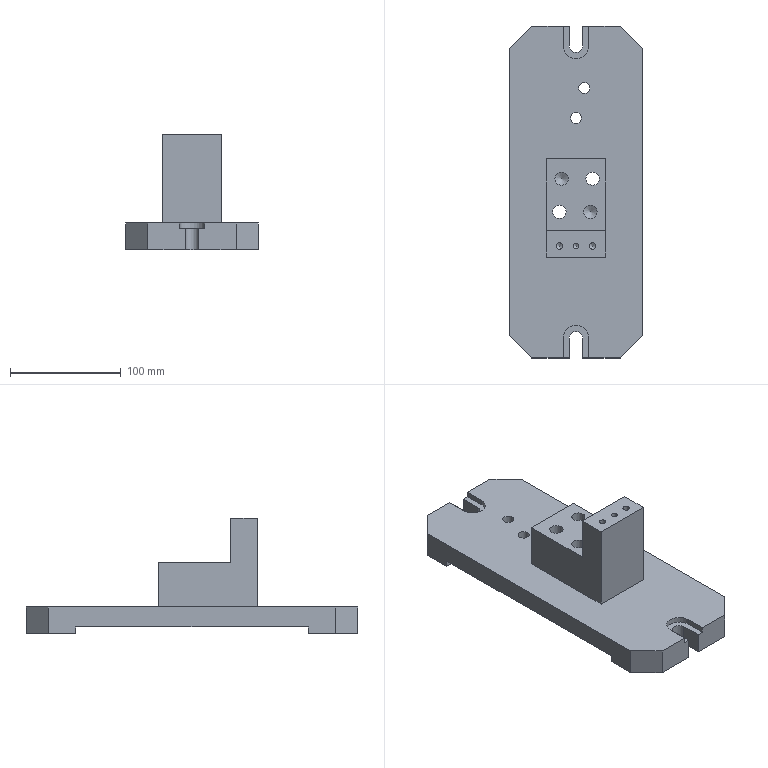Component | NX | FIXTURE_BODY | 1 solid | 51 faces | volume 899907 mm3 | plane 33 | cylinder 13 | cone 5 | commonest cylinder face diameters 12 x6 10 x2 23 x2 5.795 x2 5 x1